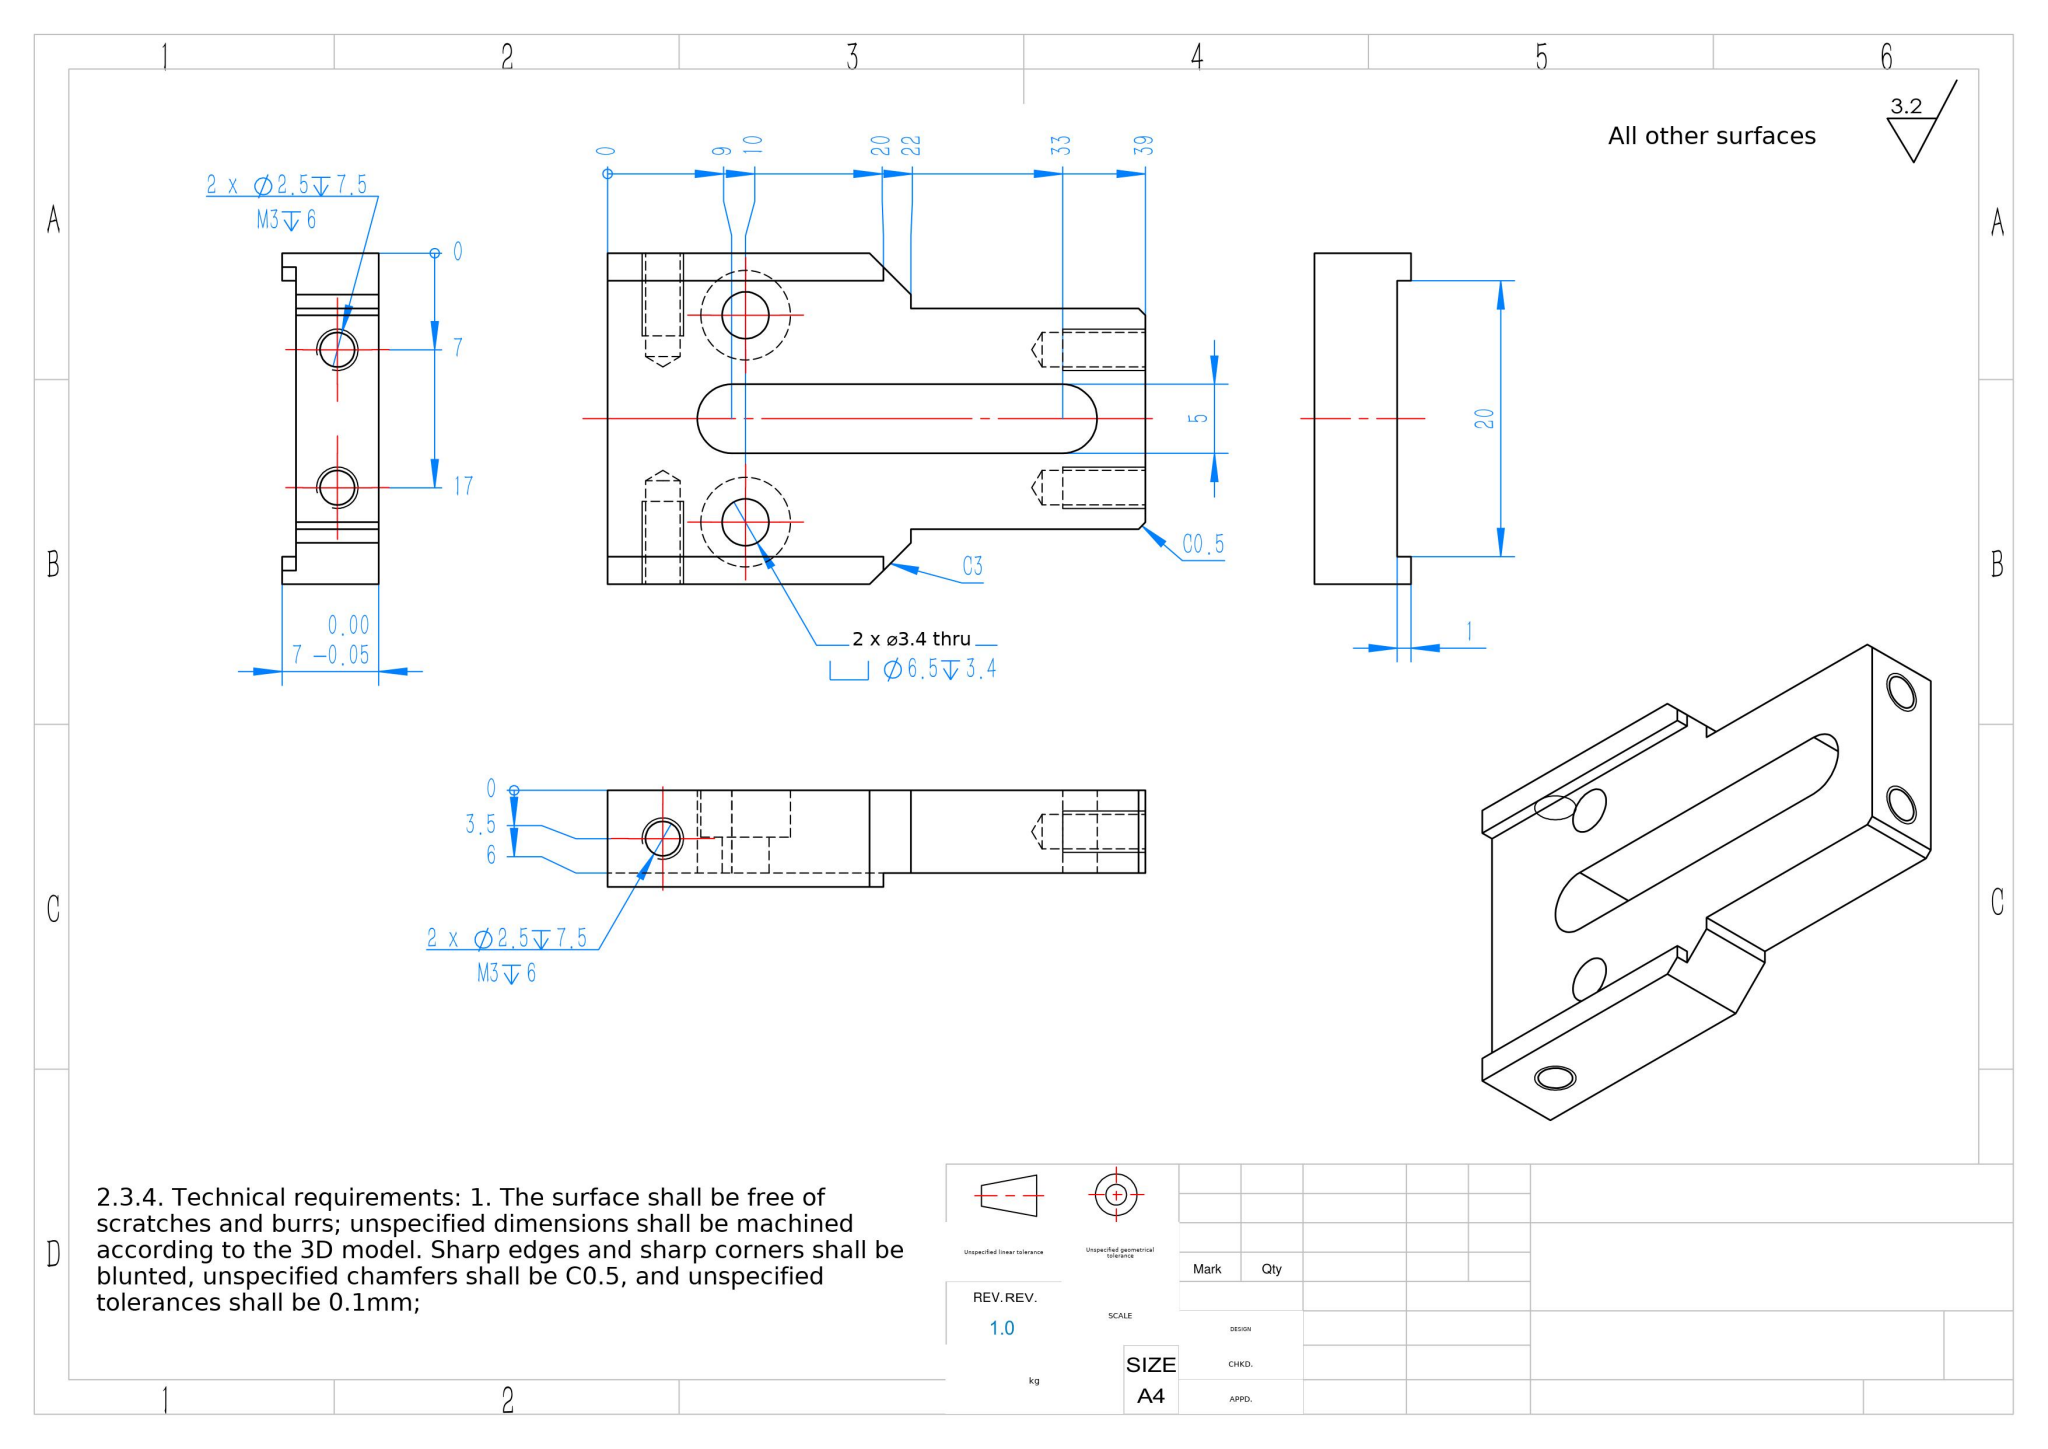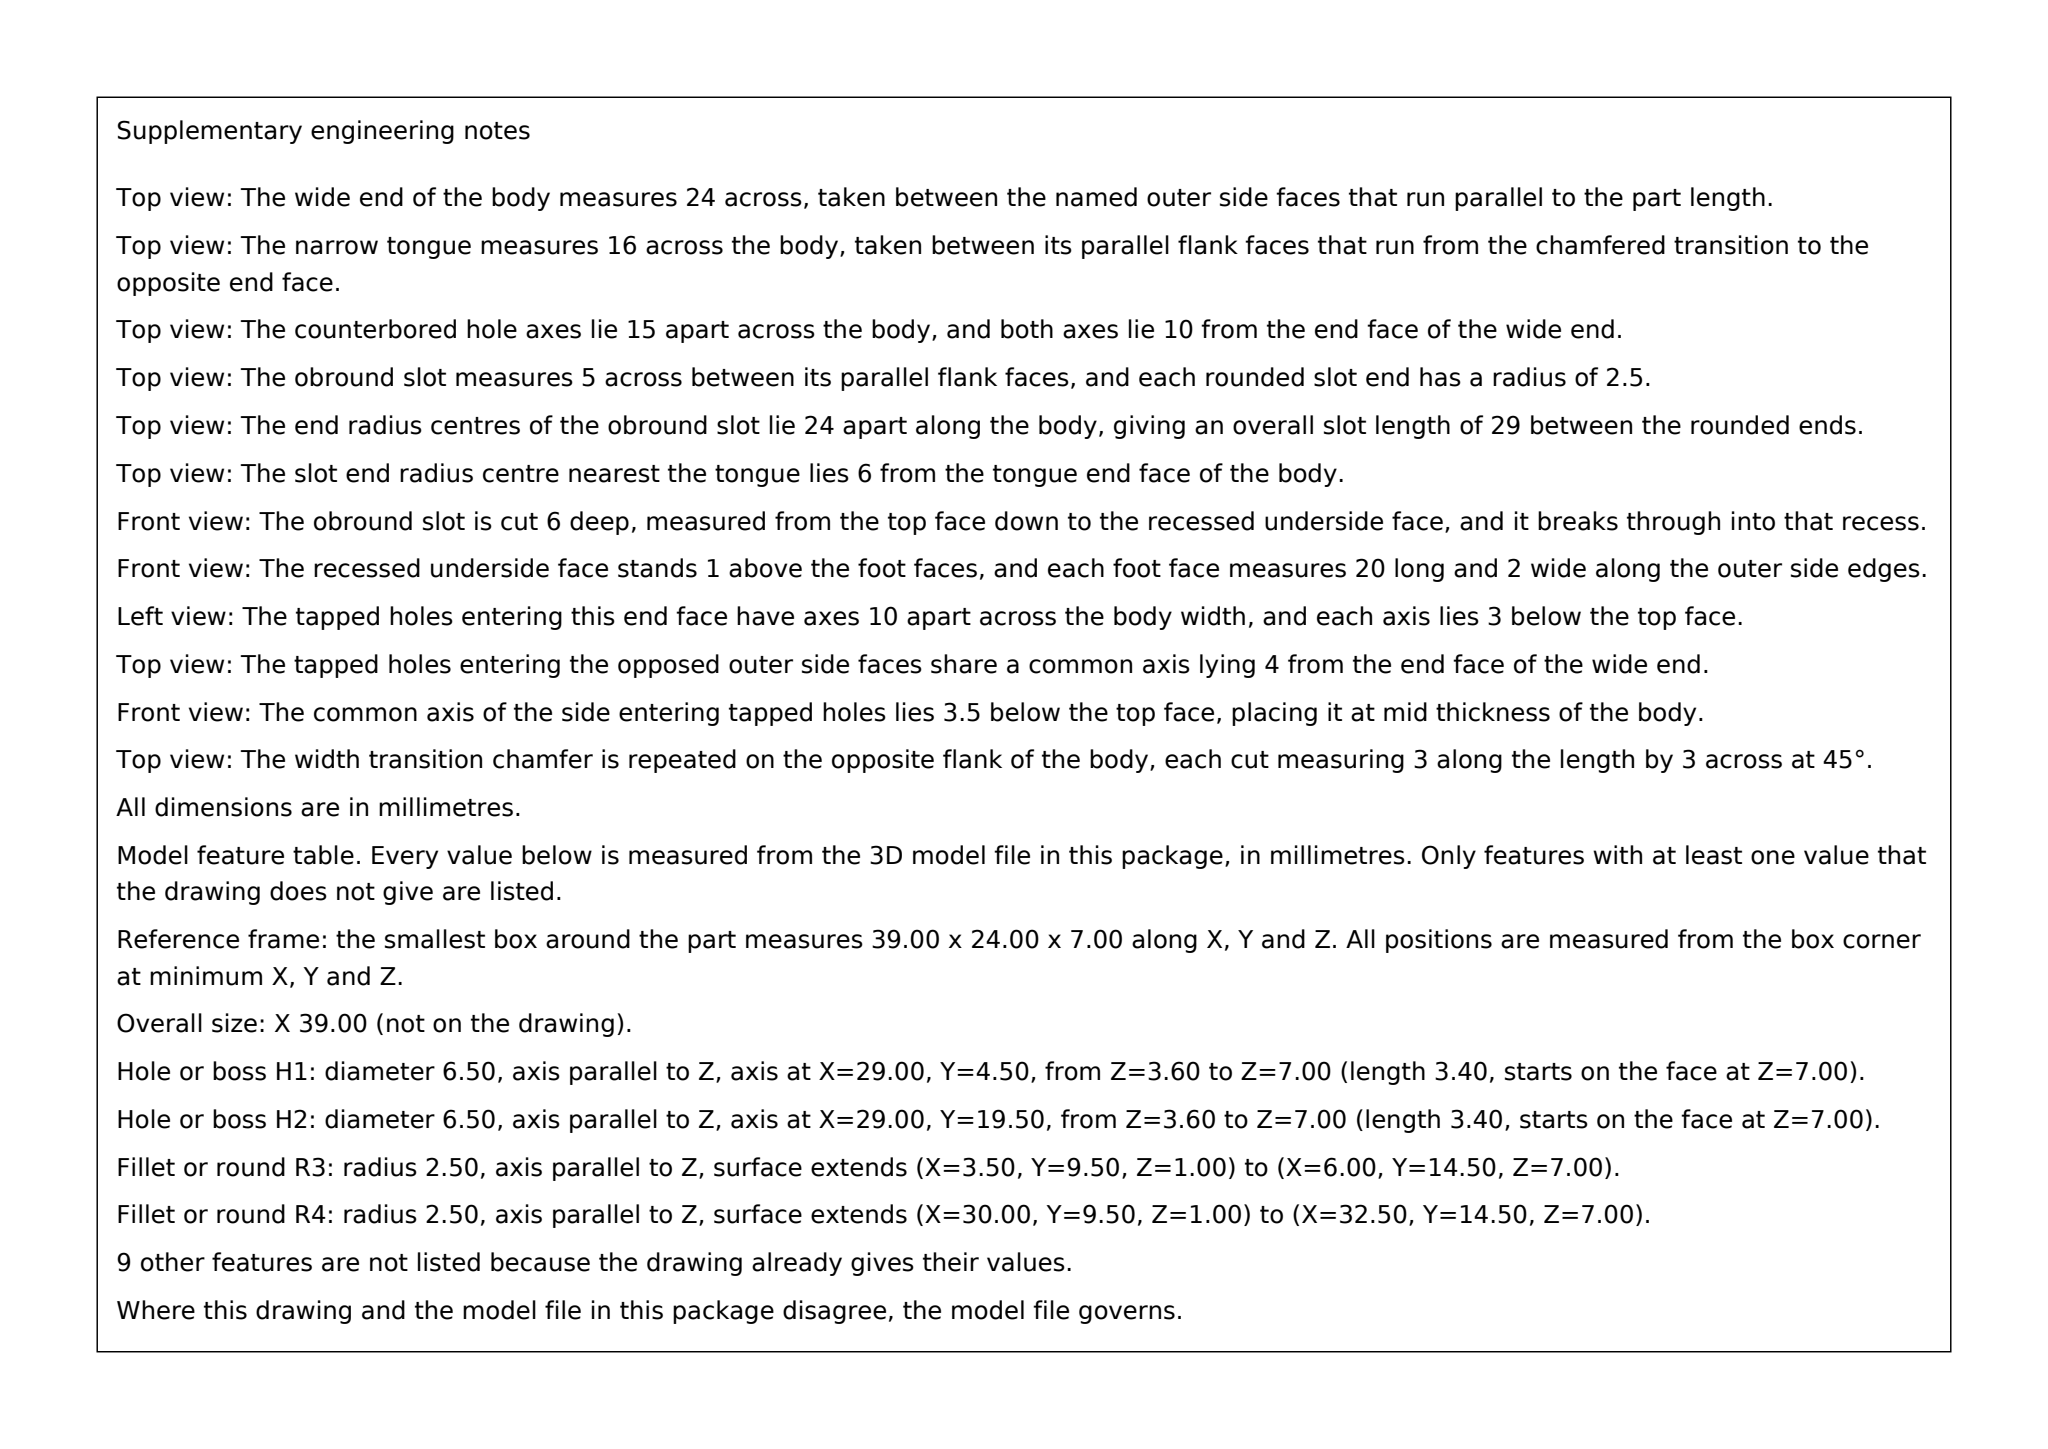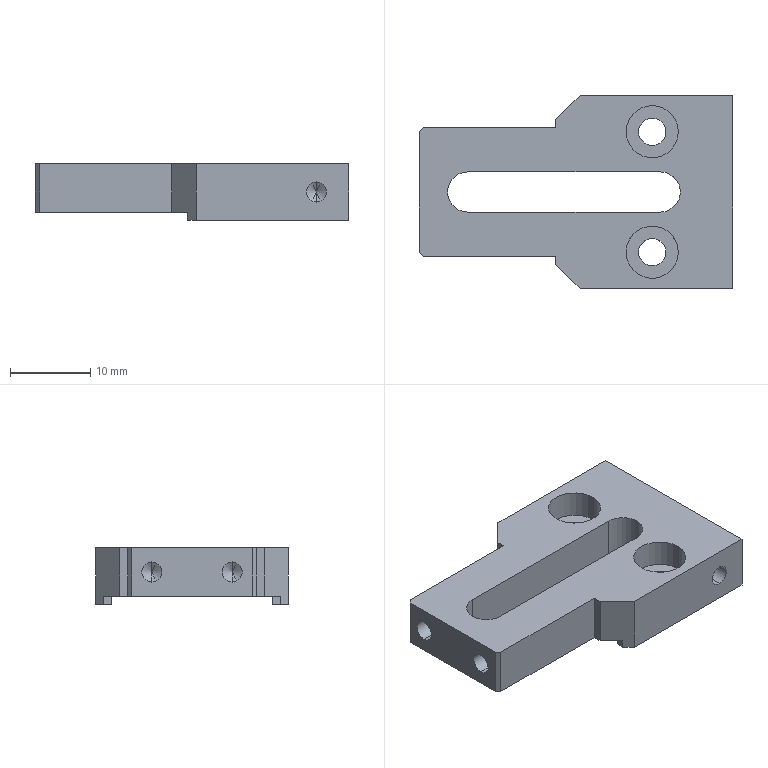Part | SolidWorks | mm | 1 solid | 51 faces | box 39 x 24 x 7 mm | volume 3561 mm3 | plane 24 | cylinder 19 | cone 8 | commonest cylinder face diameters 2.5 x8 6.5 x4 3.4 x4 5 x3
Drawing notes:
RIGHT SIDE VIEW: OVERALL 24 WIDE; 20 STEP CTRD, 2 EA SIDE | from the solid: bbox_xyz Y=24; y-planes at 0, 2, 20, 22, 24 -> 20 wide step with 2 offsets
TOP VIEW: 2X C'BORED HOLES 15 APART, SYM ABT HORIZ CL | from the solid: Ø3.4/Ø6.5 holes at y=4.5 and y=19.5 (15 apart, sym about y=12 of 24)
TOP VIEW: FORK/TONGUE END 16 WIDE, SYM ABT HORIZ CL | from the solid: y-planes 4.0 and 20.0 at RH end -> 16 wide, centered on y=12
BOTTOM VIEW: 2X M3 IN END FACE, AXES 4 FROM RH END | from the solid: Ø2.5 y-axis holes at x=35; bbox X=39 -> 39-35=4
2X M3 SIDE HOLES: AXES 3 FROM TOP FACE, 4 FROM BTM FACE | from the solid: Ø2.5 x-axis holes at z=4.0; part thk 7 (z-planes 0 and 7)
build123d program:
from build123d import *

# Parameters (mm, degrees)
SKETCH1_W                                       = 39
SKETCH1_H                                       = 24
BOSS_EXTRUDE1_DEPTH                             = 3.5
SKETCH2_W                                       = 2
SKETCH2_H                                       = 20
CUT_EXTRUDE1_DEPTH                              = 41.954
M3_HEX_SOCKET_HEAD_CAP_SCREW_CBORE1_D           = 3.4
M3_HEX_SOCKET_HEAD_CAP_SCREW_CBORE1_CBORE_D     = 6.5
M3_HEX_SOCKET_HEAD_CAP_SCREW_CBORE1_CBORE_DEPTH = 3.4
SKETCH6_W                                       = 19
SKETCH6_H                                       = 1
CUT_EXTRUDE2_DEPTH                              = 32.121
CUT_EXTRUDE4_DEPTH                              = 24.67
SKETCH15_W                                      = 17
SKETCH15_H                                      = 4
CUT_EXTRUDE5_DEPTH                              = 24.67
M3_TAPPED_HOLE1_D                               = 2.5
M3_TAPPED_HOLE1_DEPTH                           = 7.5
M3_TAPPED_HOLE1_TIP                             = 0.7511
CHAMFER1_SIZE                                   = 3
CHAMFER2_SIZE                                   = 0.5


with BuildPart() as part:
    # Sketch1 → Boss-Extrude1 (new, symmetric)
    with BuildSketch(Plane.XY):
        Rectangle(SKETCH1_W, SKETCH1_H)
    extrude(amount=BOSS_EXTRUDE1_DEPTH, both=True)

    # Sketch2 → Cut-Extrude1 (cut, through all)
    with BuildSketch(Plane.ZY.offset(19.5)):
        with Locations((-3.5, 0)):
            Rectangle(SKETCH2_W, SKETCH2_H)
    extrude(amount=-CUT_EXTRUDE1_DEPTH, mode=Mode.SUBTRACT)

    # M3 Hex Socket Head Cap Screw CBORE1 (through all)
    with Locations(Plane.XY.offset(3.5)):
        with Locations((9.5, 7.5), (9.5, -7.5)):
            CounterBoreHole(M3_HEX_SOCKET_HEAD_CAP_SCREW_CBORE1_D / 2, M3_HEX_SOCKET_HEAD_CAP_SCREW_CBORE1_CBORE_D / 2, M3_HEX_SOCKET_HEAD_CAP_SCREW_CBORE1_CBORE_DEPTH)

    # Sketch6 → Cut-Extrude2 (cut, through all)
    with BuildSketch(Plane(origin=(0, 12, 0), x_dir=(1, 0, 0), z_dir=(0, 1, 0))):
        with Locations((-10, 3)):
            Rectangle(SKETCH6_W, SKETCH6_H)
    extrude(amount=-CUT_EXTRUDE2_DEPTH, mode=Mode.SUBTRACT)

    # Sketch13 → Cut-Extrude4 (cut, through all)
    with BuildSketch(Plane(origin=(0, 0, -2.5), x_dir=(-1, 0, 0), z_dir=(0, 0, -1))):
        with BuildLine():
            Line((13.5, -2.5), (-10.5, -2.5))
            ThreePointArc((-10.5, -2.5), (-13, 0), (-10.5, 2.5))
            Line((-10.5, 2.5), (13.5, 2.5))
            ThreePointArc((13.5, 2.5), (16, 0), (13.5, -2.5))
        make_face()
    extrude(amount=-CUT_EXTRUDE4_DEPTH, mode=Mode.SUBTRACT)

    # Sketch15 → Cut-Extrude5 (cut, through all)
    with BuildSketch(Plane(origin=(0, 0, -2.5), x_dir=(-1, 0, 0), z_dir=(0, 0, -1))):
        with Locations((11, -10)):
            Rectangle(SKETCH15_W, SKETCH15_H)
        with Locations((11, 10)):
            Rectangle(SKETCH15_W, SKETCH15_H)
    extrude(amount=-CUT_EXTRUDE5_DEPTH, mode=Mode.SUBTRACT)

    # M3 Tapped Hole1
    with Locations(Plane.ZY.offset(19.5)):
        with Locations((0.5, -5), (0.5, 5)):
            Hole(M3_TAPPED_HOLE1_D / 2, depth=M3_TAPPED_HOLE1_DEPTH)
            with Locations((0, 0, -(M3_TAPPED_HOLE1_DEPTH + M3_TAPPED_HOLE1_TIP / 2))):  # 118° drill point
                Cone(0, M3_TAPPED_HOLE1_D / 2, M3_TAPPED_HOLE1_TIP, mode=Mode.SUBTRACT)

    # Chamfer1
    chamfer1_edges = [part.edges().sort_by_distance(p)[0] for p in [
        (-2.5, 12, 0.5),
        (-2.5, -12, 0.5),
    ]]
    chamfer(chamfer1_edges, length=CHAMFER1_SIZE)

    # Sketch21 → M3 Tapped Hole2 (revolve, cut)
    with BuildSketch(Plane(origin=(15.5, 12, 0), x_dir=(0, 0, 1), z_dir=(1, 0, 0))):
        Polygon((0, 0), (0, 8.251), (1.25, 7.5), (1.25, 0), align=None)
    m3_tapped_hole2 = revolve(axis=Axis((15.5, 18.35, 0), (0, -1, 0)), mode=Mode.SUBTRACT)

    # Mirror1: M3 Tapped Hole2 across plane
    add(m3_tapped_hole2.mirror(Plane.ZX), mode=Mode.SUBTRACT)

    # Chamfer2
    chamfer2_edges = [part.edges().sort_by_distance(p)[0] for p in [
        (-19.5, -8, 0.5),
        (-19.5, 8, 0.5),
    ]]
    chamfer(chamfer2_edges, length=CHAMFER2_SIZE)


solid = part.part